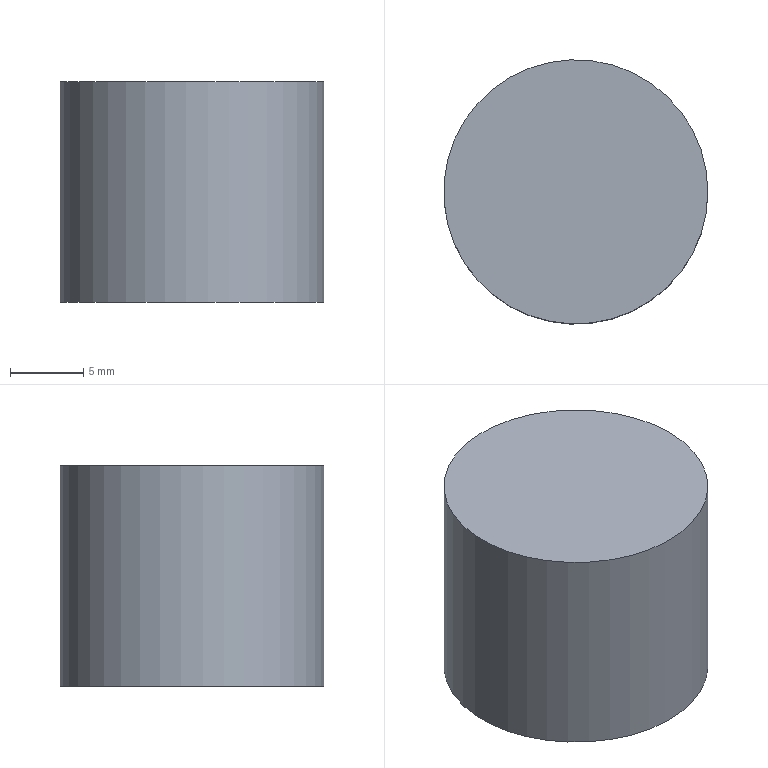Component | NX | PLUG | 1 solid | 3 faces | box 18 x 18 x 15 mm | volume 3817 mm3 | plane 2 | cylinder 1 | commonest cylinder face diameters 18 x1
STEP:
#1=CARTESIAN_POINT('',(0.,0.,0.));
#2=DIRECTION('',(0.,0.,1.));
#3=DIRECTION('',(1.,0.,0.));
#4=AXIS2_PLACEMENT_3D('',#1,#2,#3);
#5=CARTESIAN_POINT('',(3.068,1.139,53.134));
#6=VERTEX_POINT('',#5);
#7=CARTESIAN_POINT('',(-5.932,1.139,53.134));
#8=DIRECTION('',(0.,0.,-1.));
#9=DIRECTION('',(1.,0.,0.));
#10=AXIS2_PLACEMENT_3D('',#7,#8,#9);
#11=CIRCLE('',#10,9.);
#12=CARTESIAN_POINT('',(-5.932,1.139,53.134));
#13=DIRECTION('',(0.,0.,1.));
#14=DIRECTION('',(1.,0.,0.));
#15=AXIS2_PLACEMENT_3D('',#12,#13,#14);
#16=PLANE('',#15);
#17=CARTESIAN_POINT('',(9.,0.));
#18=CARTESIAN_POINT('',(9.,-15.588));
#19=CARTESIAN_POINT('',(-4.5,-7.794));
#20=CARTESIAN_POINT('',(-18.,-0.));
#21=CARTESIAN_POINT('',(-4.5,7.794));
#22=CARTESIAN_POINT('',(9.,15.588));
#23=CARTESIAN_POINT('',(9.,0.));
#24=(BOUNDED_CURVE()B_SPLINE_CURVE(2,(#17,#18,#19,#20,#21,#22,#23),.UNSPECIFIED.,.T.,.F.)B_SPLINE_CURVE_WITH_KNOTS((1,2,2,2,2,1),(-2.094,0.,2.094,4.189,6.283,8.378),.UNSPECIFIED.)CURVE()GEOMETRIC_REPRESENTATION_ITEM()RATIONAL_B_SPLINE_CURVE((1.,0.5,1.,0.5,1.,0.5,1.))REPRESENTATION_ITEM(''));
#25=(GEOMETRIC_REPRESENTATION_CONTEXT(2)PARAMETRIC_REPRESENTATION_CONTEXT()REPRESENTATION_CONTEXT('',''));
#26=DEFINITIONAL_REPRESENTATION('',(#24),#25);
#27=PCURVE('',#16,#26);
#28=CARTESIAN_POINT('',(-5.932,1.139,38.134));
#29=DIRECTION('',(0.,0.,1.));
#30=DIRECTION('',(1.,0.,0.));
#31=AXIS2_PLACEMENT_3D('',#28,#29,#30);
#32=CYLINDRICAL_SURFACE('',#31,9.);
#33=CARTESIAN_POINT('',(6.283,15.));
#34=DIRECTION('',(-1.,0.));
#35=VECTOR('',#34,1.);
#36=LINE('',#33,#35);
#37=(GEOMETRIC_REPRESENTATION_CONTEXT(2)PARAMETRIC_REPRESENTATION_CONTEXT()REPRESENTATION_CONTEXT('',''));
#38=DEFINITIONAL_REPRESENTATION('',(#36),#37);
#39=PCURVE('',#32,#38);
#40=SURFACE_CURVE('',#11,(#27,#39),.PCURVE_S1.);
#41=EDGE_CURVE('',#6,#6,#40,.T.);
#42=ORIENTED_EDGE('',*,*,#41,.F.);
#43=EDGE_LOOP('',(#42));
#44=FACE_BOUND('',#43,.T.);
#45=ADVANCED_FACE('',(#44),#16,.T.);
#46=CARTESIAN_POINT('',(3.068,1.139,38.134));
#47=VERTEX_POINT('',#46);
#48=CARTESIAN_POINT('',(-5.932,1.139,38.134));
#49=DIRECTION('',(0.,0.,1.));
#50=DIRECTION('',(1.,0.,0.));
#51=AXIS2_PLACEMENT_3D('',#48,#49,#50);
#52=CIRCLE('',#51,9.);
#53=CARTESIAN_POINT('',(-5.932,1.139,38.134));
#54=DIRECTION('',(0.,0.,-1.));
#55=DIRECTION('',(-1.,0.,0.));
#56=AXIS2_PLACEMENT_3D('',#53,#54,#55);
#57=PLANE('',#56);
#58=CARTESIAN_POINT('',(-9.,0.));
#59=CARTESIAN_POINT('',(-9.,15.588));
#60=CARTESIAN_POINT('',(4.5,7.794));
#61=CARTESIAN_POINT('',(18.,0.));
#62=CARTESIAN_POINT('',(4.5,-7.794));
#63=CARTESIAN_POINT('',(-9.,-15.588));
#64=CARTESIAN_POINT('',(-9.,0.));
#65=(BOUNDED_CURVE()B_SPLINE_CURVE(2,(#58,#59,#60,#61,#62,#63,#64),.UNSPECIFIED.,.T.,.F.)B_SPLINE_CURVE_WITH_KNOTS((1,2,2,2,2,1),(-2.094,0.,2.094,4.189,6.283,8.378),.UNSPECIFIED.)CURVE()GEOMETRIC_REPRESENTATION_ITEM()RATIONAL_B_SPLINE_CURVE((1.,0.5,1.,0.5,1.,0.5,1.))REPRESENTATION_ITEM(''));
#66=(GEOMETRIC_REPRESENTATION_CONTEXT(2)PARAMETRIC_REPRESENTATION_CONTEXT()REPRESENTATION_CONTEXT('',''));
#67=DEFINITIONAL_REPRESENTATION('',(#65),#66);
#68=PCURVE('',#57,#67);
#69=CARTESIAN_POINT('',(0.,0.));
#70=DIRECTION('',(1.,0.));
#71=VECTOR('',#70,1.);
#72=LINE('',#69,#71);
#73=(GEOMETRIC_REPRESENTATION_CONTEXT(2)PARAMETRIC_REPRESENTATION_CONTEXT()REPRESENTATION_CONTEXT('',''));
#74=DEFINITIONAL_REPRESENTATION('',(#72),#73);
#75=PCURVE('',#32,#74);
#76=SURFACE_CURVE('',#52,(#68,#75),.PCURVE_S1.);
#77=EDGE_CURVE('',#47,#47,#76,.T.);
#78=ORIENTED_EDGE('',*,*,#77,.F.);
#79=EDGE_LOOP('',(#78));
#80=FACE_BOUND('',#79,.T.);
#81=ADVANCED_FACE('',(#80),#57,.T.);
#82=ORIENTED_EDGE('',*,*,#41,.T.);
#83=CARTESIAN_POINT('',(3.068,1.139,38.134));
#84=CARTESIAN_POINT('',(3.068,1.139,53.134));
#85=B_SPLINE_CURVE_WITH_KNOTS('',1,(#83,#84),.UNSPECIFIED.,.F.,.F.,(2,2),(0.,15.),.PIECEWISE_BEZIER_KNOTS.);
#86=CARTESIAN_POINT('',(0.,0.));
#87=DIRECTION('',(0.,1.));
#88=VECTOR('',#87,1.);
#89=LINE('',#86,#88);
#90=(GEOMETRIC_REPRESENTATION_CONTEXT(2)PARAMETRIC_REPRESENTATION_CONTEXT()REPRESENTATION_CONTEXT('',''));
#91=DEFINITIONAL_REPRESENTATION('',(#89),#90);
#92=PCURVE('',#32,#91);
#93=CARTESIAN_POINT('',(6.283,0.));
#94=DIRECTION('',(0.,1.));
#95=VECTOR('',#94,1.);
#96=LINE('',#93,#95);
#97=(GEOMETRIC_REPRESENTATION_CONTEXT(2)PARAMETRIC_REPRESENTATION_CONTEXT()REPRESENTATION_CONTEXT('',''));
#98=DEFINITIONAL_REPRESENTATION('',(#96),#97);
#99=PCURVE('',#32,#98);
#100=SEAM_CURVE('',#85,(#92,#99),.PCURVE_S1.);
#101=EDGE_CURVE('',#47,#6,#100,.T.);
#102=ORIENTED_EDGE('',*,*,#101,.F.);
#103=ORIENTED_EDGE('',*,*,#77,.T.);
#104=ORIENTED_EDGE('',*,*,#101,.T.);
#105=EDGE_LOOP('',(#82,#102,#103,#104));
#106=FACE_BOUND('',#105,.T.);
#107=ADVANCED_FACE('',(#106),#32,.T.);
#108=CLOSED_SHELL('',(#45,#81,#107));
#109=MANIFOLD_SOLID_BREP('',#108);
#110=(LENGTH_UNIT()NAMED_UNIT(*)SI_UNIT(.MILLI.,.METRE.));
#111=UNCERTAINTY_MEASURE_WITH_UNIT(LENGTH_MEASURE(0.00001),#110,'','');
#112=(NAMED_UNIT(*)PLANE_ANGLE_UNIT()SI_UNIT($,.RADIAN.));
#113=(NAMED_UNIT(*)SI_UNIT($,.STERADIAN.)SOLID_ANGLE_UNIT());
#114=(GEOMETRIC_REPRESENTATION_CONTEXT(3)GLOBAL_UNCERTAINTY_ASSIGNED_CONTEXT((#111))GLOBAL_UNIT_ASSIGNED_CONTEXT((#110,#112,#113))REPRESENTATION_CONTEXT('',''));
#115=ADVANCED_BREP_SHAPE_REPRESENTATION('',(#4,#109),#114);